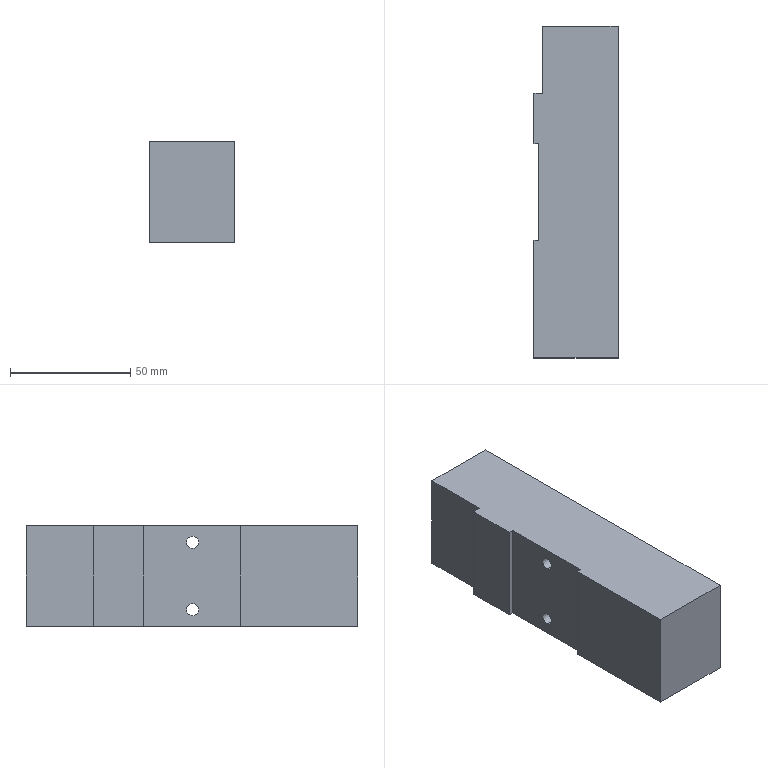Component | SolidWorks | SuctionCupMountingBlock(Fixed)-1 | 1 solid | 33 faces | box 35 x 138 x 42 mm | volume 178895 mm3 | cylinder 20 | plane 13 | commonest cylinder face diameters 6 x14 5 x4 12 x2
build123d program:
from build123d import *

# Parameters (mm, degrees)
SKETCH2_W           = 35
SKETCH2_H           = 138
BOSS_EXTRUDE1_DEPTH = 42
SKETCH3_R           = 3
CUT_EXTRUDE1_DEPTH  = 14
SKETCH4_R           = 6
CUT_EXTRUDE2_DEPTH  = 120
SKETCH5_W           = 2
SKETCH5_H           = 40
CUT_EXTRUDE3_DEPTH  = 42
M6_TAPPED_HOLE1_D   = 5
SKETCH8_W           = 3.5
SKETCH8_H           = 28
CUT_EXTRUDE4_DEPTH  = 53


with BuildPart() as part:
    # Sketch2 → Boss-Extrude1 (new body)
    with BuildSketch(Plane.XY):
        with Locations((17.731, -60.264)):
            Rectangle(SKETCH2_W, SKETCH2_H)
    extrude(amount=-BOSS_EXTRUDE1_DEPTH)

    # Sketch3 → Cut-Extrude1 (cut)
    with BuildSketch(Plane.ZY.offset(-0.2307)):
        with Locations(Location((-21, -3.264, 0), (0, 0, 270))):
            Circle(SKETCH3_R)
        with Locations(Location((-21, -75.264, 0), (0, 0, 270))):
            Circle(SKETCH3_R)
        with Locations(Location((-21, -18.264, 0), (0, 0, 270))):
            Circle(SKETCH3_R)
        with Locations(Location((-21, -33.264, 0), (0, 0, 270))):
            Circle(SKETCH3_R)
        with Locations(Location((-21, -48.264, 0), (0, 0, 270))):
            Circle(SKETCH3_R)
        with Locations(Location((-21, -90.264, 0), (0, 0, 270))):
            Circle(SKETCH3_R)
        with Locations(Location((-21, -105.264, 0), (0, 0, 270))):
            Circle(SKETCH3_R)
    extrude(amount=-CUT_EXTRUDE1_DEPTH, mode=Mode.SUBTRACT)

    # Sketch4 → Cut-Extrude2 (cut)
    with BuildSketch(Plane(origin=(0, 8.736, 0), x_dir=(1, 0, 0), z_dir=(0, 1, 0))):
        with Locations(Location((14.231, 21, 0), (0, 0, 180))):
            Circle(SKETCH4_R)
    extrude(amount=-CUT_EXTRUDE2_DEPTH, mode=Mode.SUBTRACT)

    # Sketch5 → Cut-Extrude3 (cut)
    with BuildSketch(Plane.XY):
        with Locations((34.231, -60.264)):
            Rectangle(SKETCH5_W, SKETCH5_H)
    extrude(amount=-CUT_EXTRUDE3_DEPTH, mode=Mode.SUBTRACT)

    # M6 Tapped Hole1 (through all)
    with Locations(Plane(origin=(33.231, 0, 0), x_dir=(0, 0, -1), z_dir=(1, 0, 0))):
        with Locations((7, -60.514), (35, -60.514)):
            Hole(M6_TAPPED_HOLE1_D / 2)

    # Sketch8 → Cut-Extrude4 (cut)
    with BuildSketch(Plane.XY):
        with Locations((33.481, -5.264)):
            Rectangle(SKETCH8_W, SKETCH8_H)
    extrude(amount=-CUT_EXTRUDE4_DEPTH, mode=Mode.SUBTRACT)


solid = part.part

# Placed as in the assembly
solid = solid.moved(Location((-571.465, -18.387, 352.468), (-180, 0, 180)))